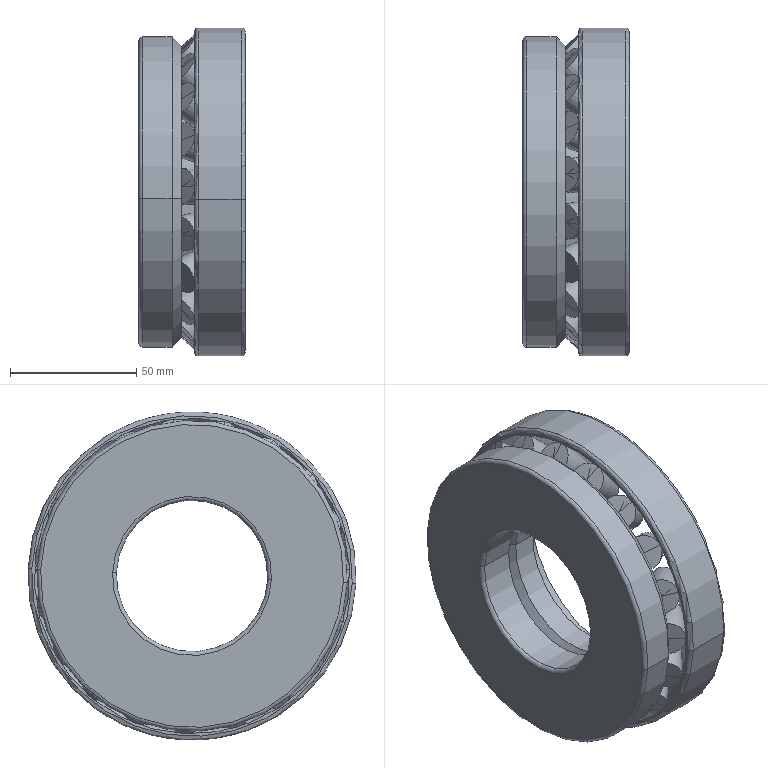Component | SolidWorks | self-aligning thrust roller bearings gb-1 | 21 solids | 131 faces | volume 318888 mm3 | torus 48 | cone 48 | plane 23 | cylinder 10 | sphere 2 | commonest cylinder face diameters 123 x2 60 x2 63 x2 89 x2 130 x2